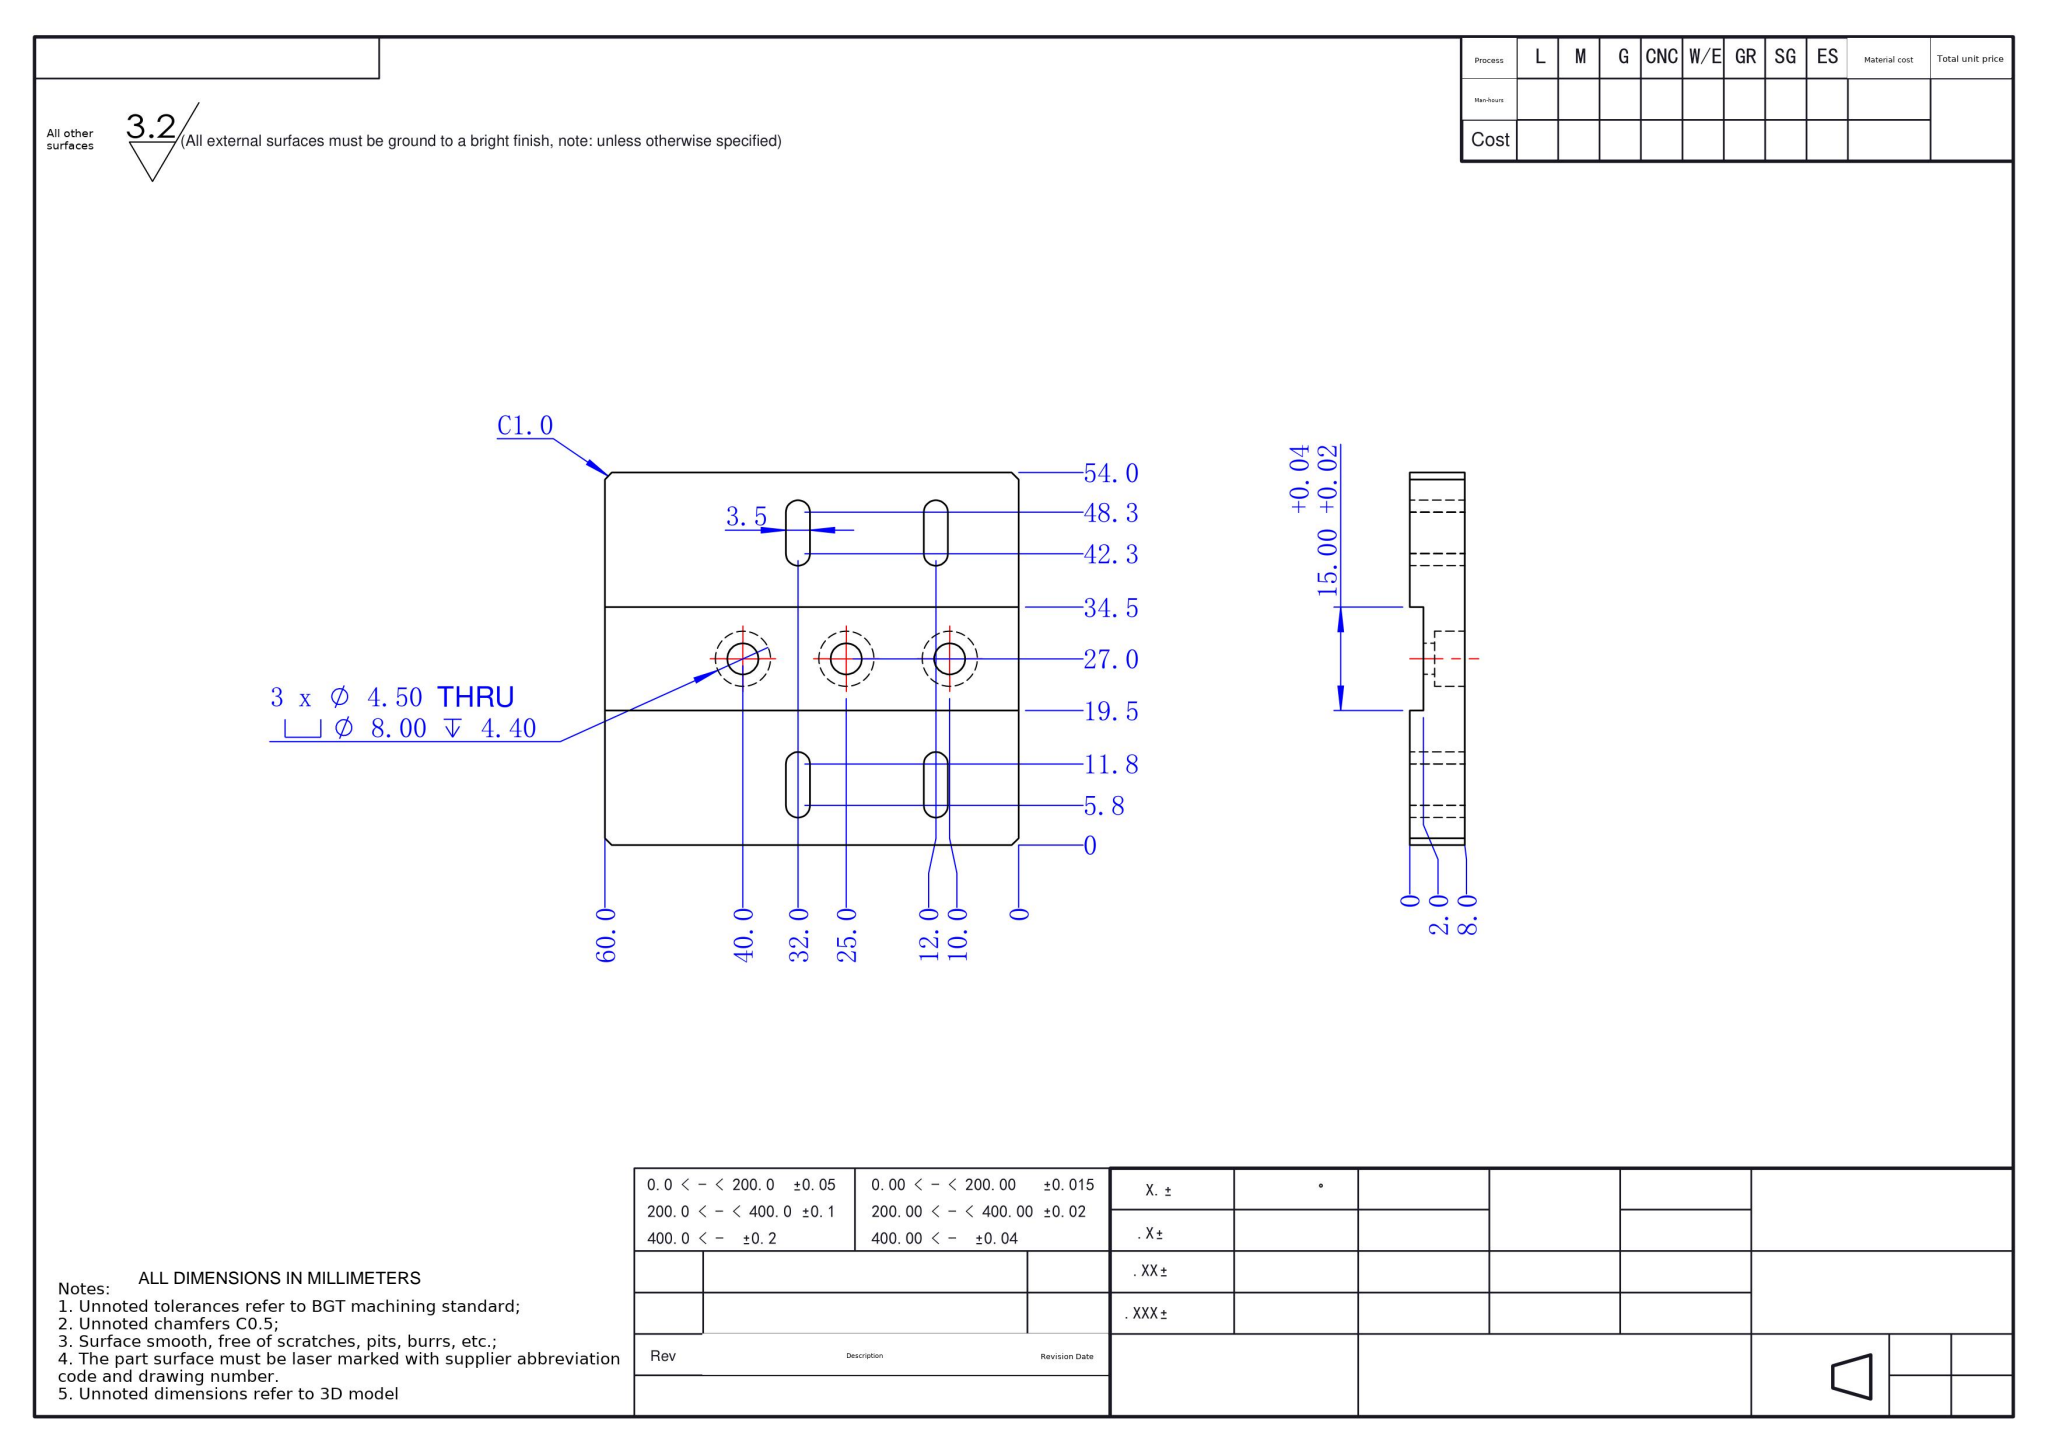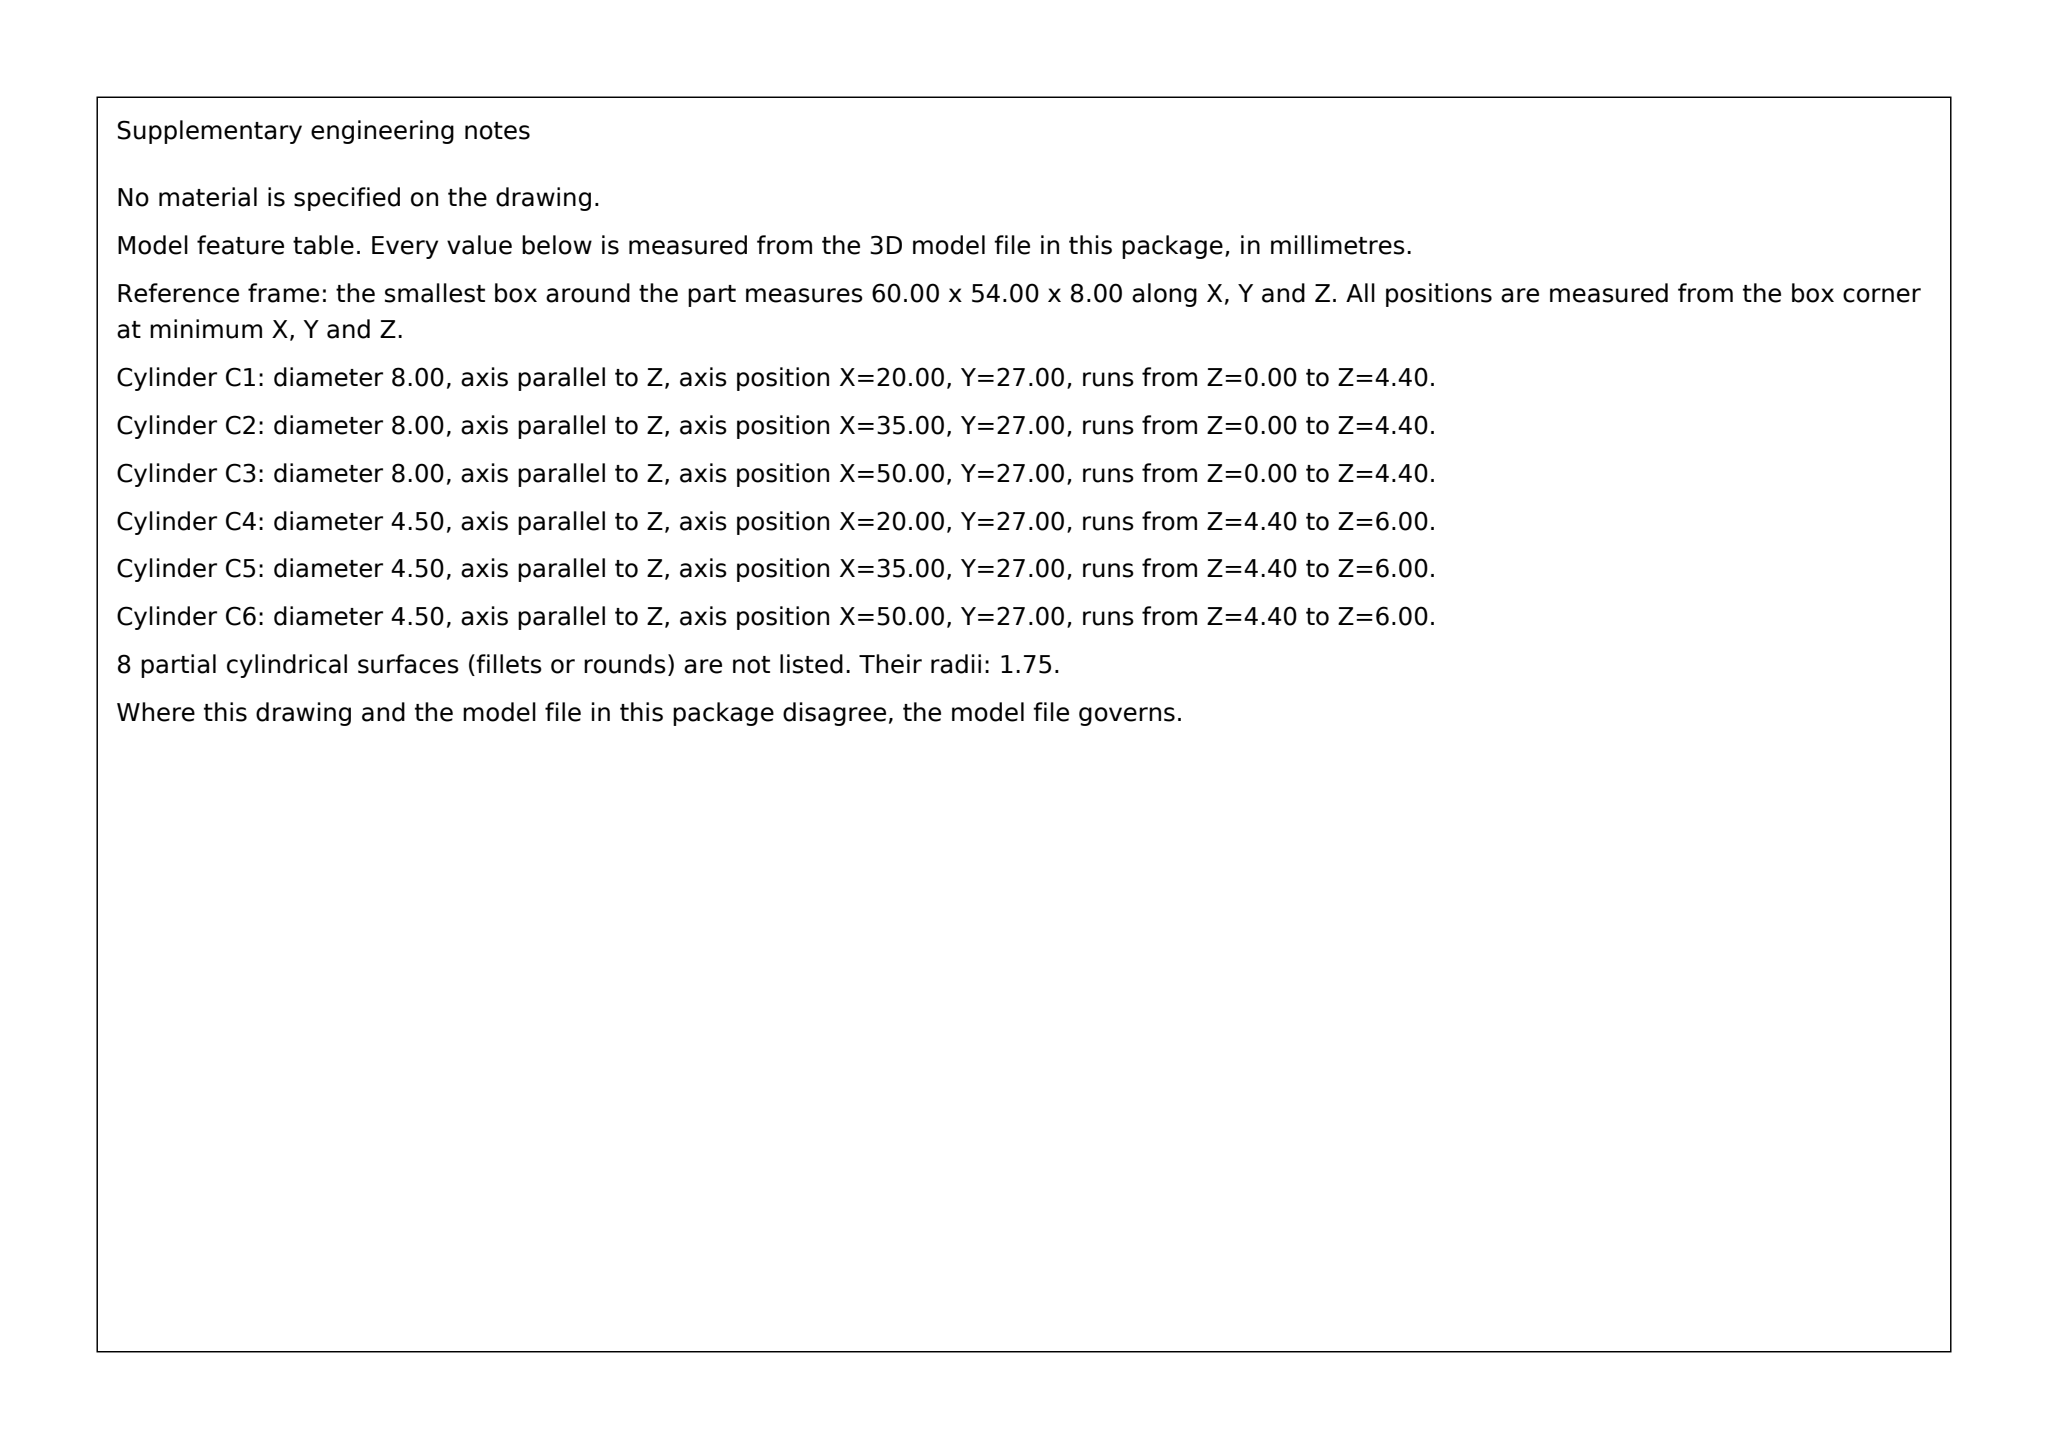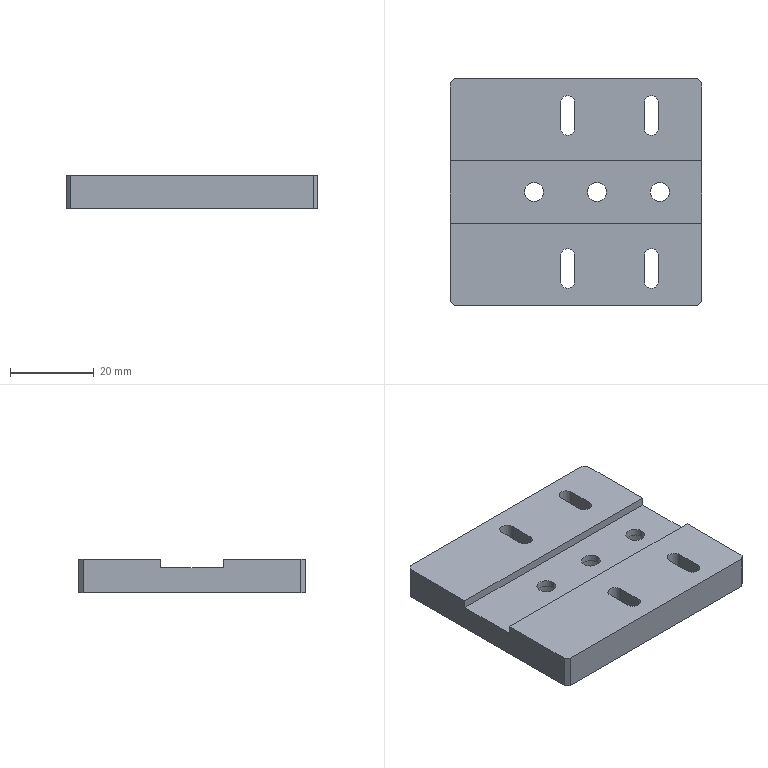Part | SolidWorks | mm | 1 solid | 45 faces | box 60 x 54 x 8 mm | volume 22384 mm3 | plane 25 | cylinder 20 | commonest cylinder face diameters 3.5 x8 8 x6 4.5 x6
build123d program:
from build123d import *

# Parameters (mm, degrees)
SKETCH1_W                                       = 60
SKETCH1_H                                       = 54
BOSS_EXTRUDE1_DEPTH                             = 8
F_3_5_3_5_DIAMETER_HOLE1_D                      = 3.5
SKETCH4_W                                       = 60
SKETCH4_H                                       = 15
CUT_EXTRUDE1_DEPTH                              = 2
M4_HEX_SOCKET_HEAD_CAP_SCREW_CBORE1_D           = 4.5
M4_HEX_SOCKET_HEAD_CAP_SCREW_CBORE1_CBORE_D     = 8
M4_HEX_SOCKET_HEAD_CAP_SCREW_CBORE1_CBORE_DEPTH = 4.4
CHAMFER1_SIZE                                   = 1
CUT_EXTRUDE2_DEPTH                              = 82.117


with BuildPart() as part:
    # Sketch1 → Boss-Extrude1 (new body)
    with BuildSketch(Plane.XY):
        with Locations((30, 27)):
            Rectangle(SKETCH1_W, SKETCH1_H)
    extrude(amount=BOSS_EXTRUDE1_DEPTH)

    # 3.5 _3.5_ Diameter Hole1 (through all)
    with Locations(Plane(origin=(0, 0, 0), x_dir=(-1, 0, 0), z_dir=(0, 0, -1))):
        with Locations((-48, 45.25), (-28, 45.25), (-28, 8.75), (-48, 8.75)):
            Hole(F_3_5_3_5_DIAMETER_HOLE1_D / 2)

    # Sketch4 → Cut-Extrude1 (cut)
    with BuildSketch(Plane.XY.offset(8)):
        with Locations((30, 27)):
            Rectangle(SKETCH4_W, SKETCH4_H)
    extrude(amount=-CUT_EXTRUDE1_DEPTH, mode=Mode.SUBTRACT)

    # M4 Hex Socket Head Cap Screw CBORE1 (through all)
    with Locations(Plane(origin=(0, 0, 0), x_dir=(-1, 0, 0), z_dir=(0, 0, -1))):
        with Locations((-50, 27), (-35, 27), (-20, 27)):
            CounterBoreHole(M4_HEX_SOCKET_HEAD_CAP_SCREW_CBORE1_D / 2, M4_HEX_SOCKET_HEAD_CAP_SCREW_CBORE1_CBORE_D / 2, M4_HEX_SOCKET_HEAD_CAP_SCREW_CBORE1_CBORE_DEPTH)

    # Chamfer1
    chamfer1_edges = [part.edges().sort_by_distance(p)[0] for p in [
        (0, 54, 4),
        (60, 54, 4),
        (60, 0, 4),
        (0, 0, 4),
    ]]
    chamfer(chamfer1_edges, length=CHAMFER1_SIZE)

    # Sketch7 → Cut-Extrude2 (cut, through all)
    with BuildSketch(Plane(origin=(0, 0, 0), x_dir=(-1, 0, 0), z_dir=(0, 0, -1))):
        with BuildLine():
            Line((-49.75, 5.75), (-49.75, 11.75))
            ThreePointArc((-49.75, 11.75), (-48, 13.5), (-46.25, 11.75))
            Line((-46.25, 11.75), (-46.25, 5.75))
            ThreePointArc((-46.25, 5.75), (-48, 4), (-49.75, 5.75))
        make_face()
        with BuildLine():
            Line((-29.75, 5.75), (-29.75, 11.75))
            ThreePointArc((-29.75, 11.75), (-28, 13.5), (-26.25, 11.75))
            Line((-26.25, 11.75), (-26.25, 5.75))
            ThreePointArc((-26.25, 5.75), (-28, 4), (-29.75, 5.75))
        make_face()
        with BuildLine():
            Line((-49.75, 42.25), (-49.75, 48.25))
            ThreePointArc((-49.75, 48.25), (-48, 50), (-46.25, 48.25))
            Line((-46.25, 48.25), (-46.25, 42.25))
            ThreePointArc((-46.25, 42.25), (-48, 40.5), (-49.75, 42.25))
        make_face()
        with BuildLine():
            Line((-29.75, 42.25), (-29.75, 48.25))
            ThreePointArc((-29.75, 48.25), (-28, 50), (-26.25, 48.25))
            Line((-26.25, 48.25), (-26.25, 42.25))
            ThreePointArc((-26.25, 42.25), (-28, 40.5), (-29.75, 42.25))
        make_face()
    extrude(amount=-CUT_EXTRUDE2_DEPTH, mode=Mode.SUBTRACT)


solid = part.part